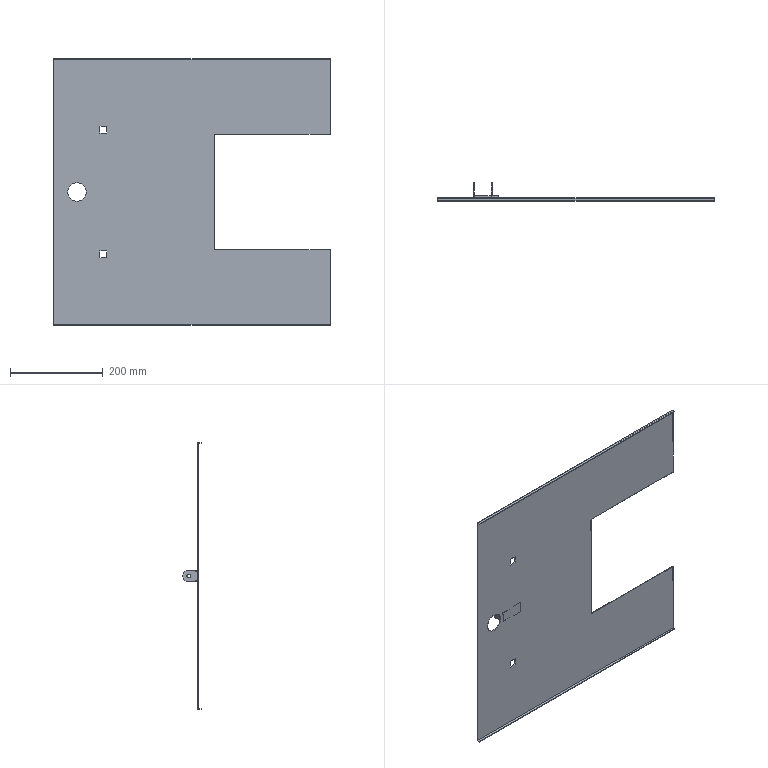Component | SolidWorks | InsectCollectionPlatform-1 | 1 solid | 43 faces | box 597 x 39 x 577 mm | volume 434724 mm3 | plane 35 | cylinder 8 | commonest cylinder face diameters 8 x4 40 x2 25 x2
build123d program:
from build123d import *

# Parameters (mm, degrees)
BOSS_EXTRUDE1_2_DEPTH = 1.5
SKETCH2_2_R           = 20
CUT_EXTRUDE1_2_DEPTH  = 1.5
SKETCH3_2_W           = 597
SKETCH3_2_H           = 6.5
BOSS_EXTRUDE2_2_DEPTH = 1.5
SKETCH1_W             = 15
SKETCH1_H             = 15
SKETCH1_R             = 7.5
CUT_EXTRUDE1_DEPTH    = 5
SKETCH2_W             = 40
SKETCH2_H             = 25
SKETCH2_W_2           = 36
SKETCH2_H_2           = 21
BOSS_EXTRUDE1_DEPTH   = 5
SKETCH3_R             = 4
BOSS_EXTRUDE2_DEPTH   = 2
SKETCH4_W             = 15
SKETCH4_H             = 25
BOSS_EXTRUDE3_DEPTH   = 5


with BuildPart() as part:
    # Sketch1_2 → Boss-Extrude1_2 (new body)
    with BuildSketch(Plane(origin=(0, 0, 0), x_dir=(1, 0, 0), z_dir=(0, 1, 0))):
        Polygon((298.5, 288.5), (-298.5, 288.5), (-298.5, -288.5), (298.5, -288.5), (298.5, -125), (48.5, -125), (48.5, 125), (298.5, 125), align=None)
    extrude(amount=BOSS_EXTRUDE1_2_DEPTH)

    # Sketch2_2 → Cut-Extrude1_2 (cut)
    with BuildSketch(Plane(origin=(0, 1.5, 0), x_dir=(1, 0, 0), z_dir=(0, 1, 0))):
        with Locations(Location((-248.5, 0, 0), (0, 0, 270))):
            Circle(SKETCH2_2_R)
    extrude(amount=-CUT_EXTRUDE1_2_DEPTH, mode=Mode.SUBTRACT)

    # Sketch3_2 → Boss-Extrude2_2 (add)
    with BuildSketch(Plane.XY.offset(288.5)):
        with Locations((0, -1.75)):
            Rectangle(SKETCH3_2_W, SKETCH3_2_H)
    boss_extrude2_2 = extrude(amount=-BOSS_EXTRUDE2_2_DEPTH)

    # Mirror1_2: Boss-Extrude2_2 across plane
    add(boss_extrude2_2.mirror(Plane.XY))

    # Sketch1 → Cut-Extrude1 (cut, symmetric)
    # profile 1 of 2: a face of its own
    with BuildSketch(Plane(origin=(0, 1.5, 0), x_dir=(1, 0, 0), z_dir=(0, 1, 0))):
        with Locations((-191.5, -135)):
            Rectangle(SKETCH1_W, SKETCH1_H)
        with Locations((-191.5, -135)):
            Circle(SKETCH1_R, mode=Mode.SUBTRACT)
    # profile 2 of 2: a face of its own
    with BuildSketch(Plane(origin=(0, 1.5, 0), x_dir=(1, 0, 0), z_dir=(0, 1, 0))):
        with Locations((-191.5, 135)):
            Rectangle(SKETCH1_W, SKETCH1_H)
        with Locations((-191.5, 135)):
            Circle(SKETCH1_R, mode=Mode.SUBTRACT)
    extrude(amount=CUT_EXTRUDE1_DEPTH, both=True, mode=Mode.SUBTRACT)


with BuildPart() as cut_extrude1_kept_piece:
    # of the separate pieces the step leaves, the one the design keeps (cut_extrude1_pieces_kept)
    add(part.part.solids().sort_by_distance((298.5, 1.5, -288.5))[0])

    # Sketch2 → Boss-Extrude1 (add)
    with BuildSketch(Plane(origin=(0, 1.5, 0), x_dir=(1, 0, 0), z_dir=(0, 1, 0))):
        with Locations((-201.5, 0)):
            Rectangle(SKETCH2_W, SKETCH2_H)
        with Locations((-201.5, 0)):
            Rectangle(SKETCH2_W_2, SKETCH2_H_2, mode=Mode.SUBTRACT)
    extrude(amount=BOSS_EXTRUDE1_DEPTH)

    # Sketch3 → Boss-Extrude2 (add)
    with BuildSketch(Plane.ZY.offset(221.5)):
        with BuildLine():
            Line((-12.5, 6.5), (-12.5, 21.5))
            ThreePointArc((-12.5, 21.5), (0, 34), (12.5, 21.5))
            Line((12.5, 21.5), (12.5, 6.5))
            Line((12.5, 6.5), (-12.5, 6.5))
        make_face()
        with Locations((0, 21.5)):
            Circle(SKETCH3_R, mode=Mode.SUBTRACT)
    boss_extrude2 = extrude(amount=-BOSS_EXTRUDE2_DEPTH)

    # Mirror1: Boss-Extrude2 across plane
    add(boss_extrude2.mirror(Plane(origin=(-201.5, 0, 0), x_dir=(0, 0, 1), z_dir=(1, 0, 0))))

    # Sketch4 → Boss-Extrude3 (add)
    with BuildSketch(Plane(origin=(0, 1.5, 0), x_dir=(1, 0, 0), z_dir=(0, 1, 0))):
        with Locations((-174, 0)):
            Rectangle(SKETCH4_W, SKETCH4_H)
    extrude(amount=BOSS_EXTRUDE3_DEPTH)


solid = cut_extrude1_kept_piece.part

# Placed as in the assembly
solid = solid.moved(Location((0, 198.5, -10), (0, 0, 0)))